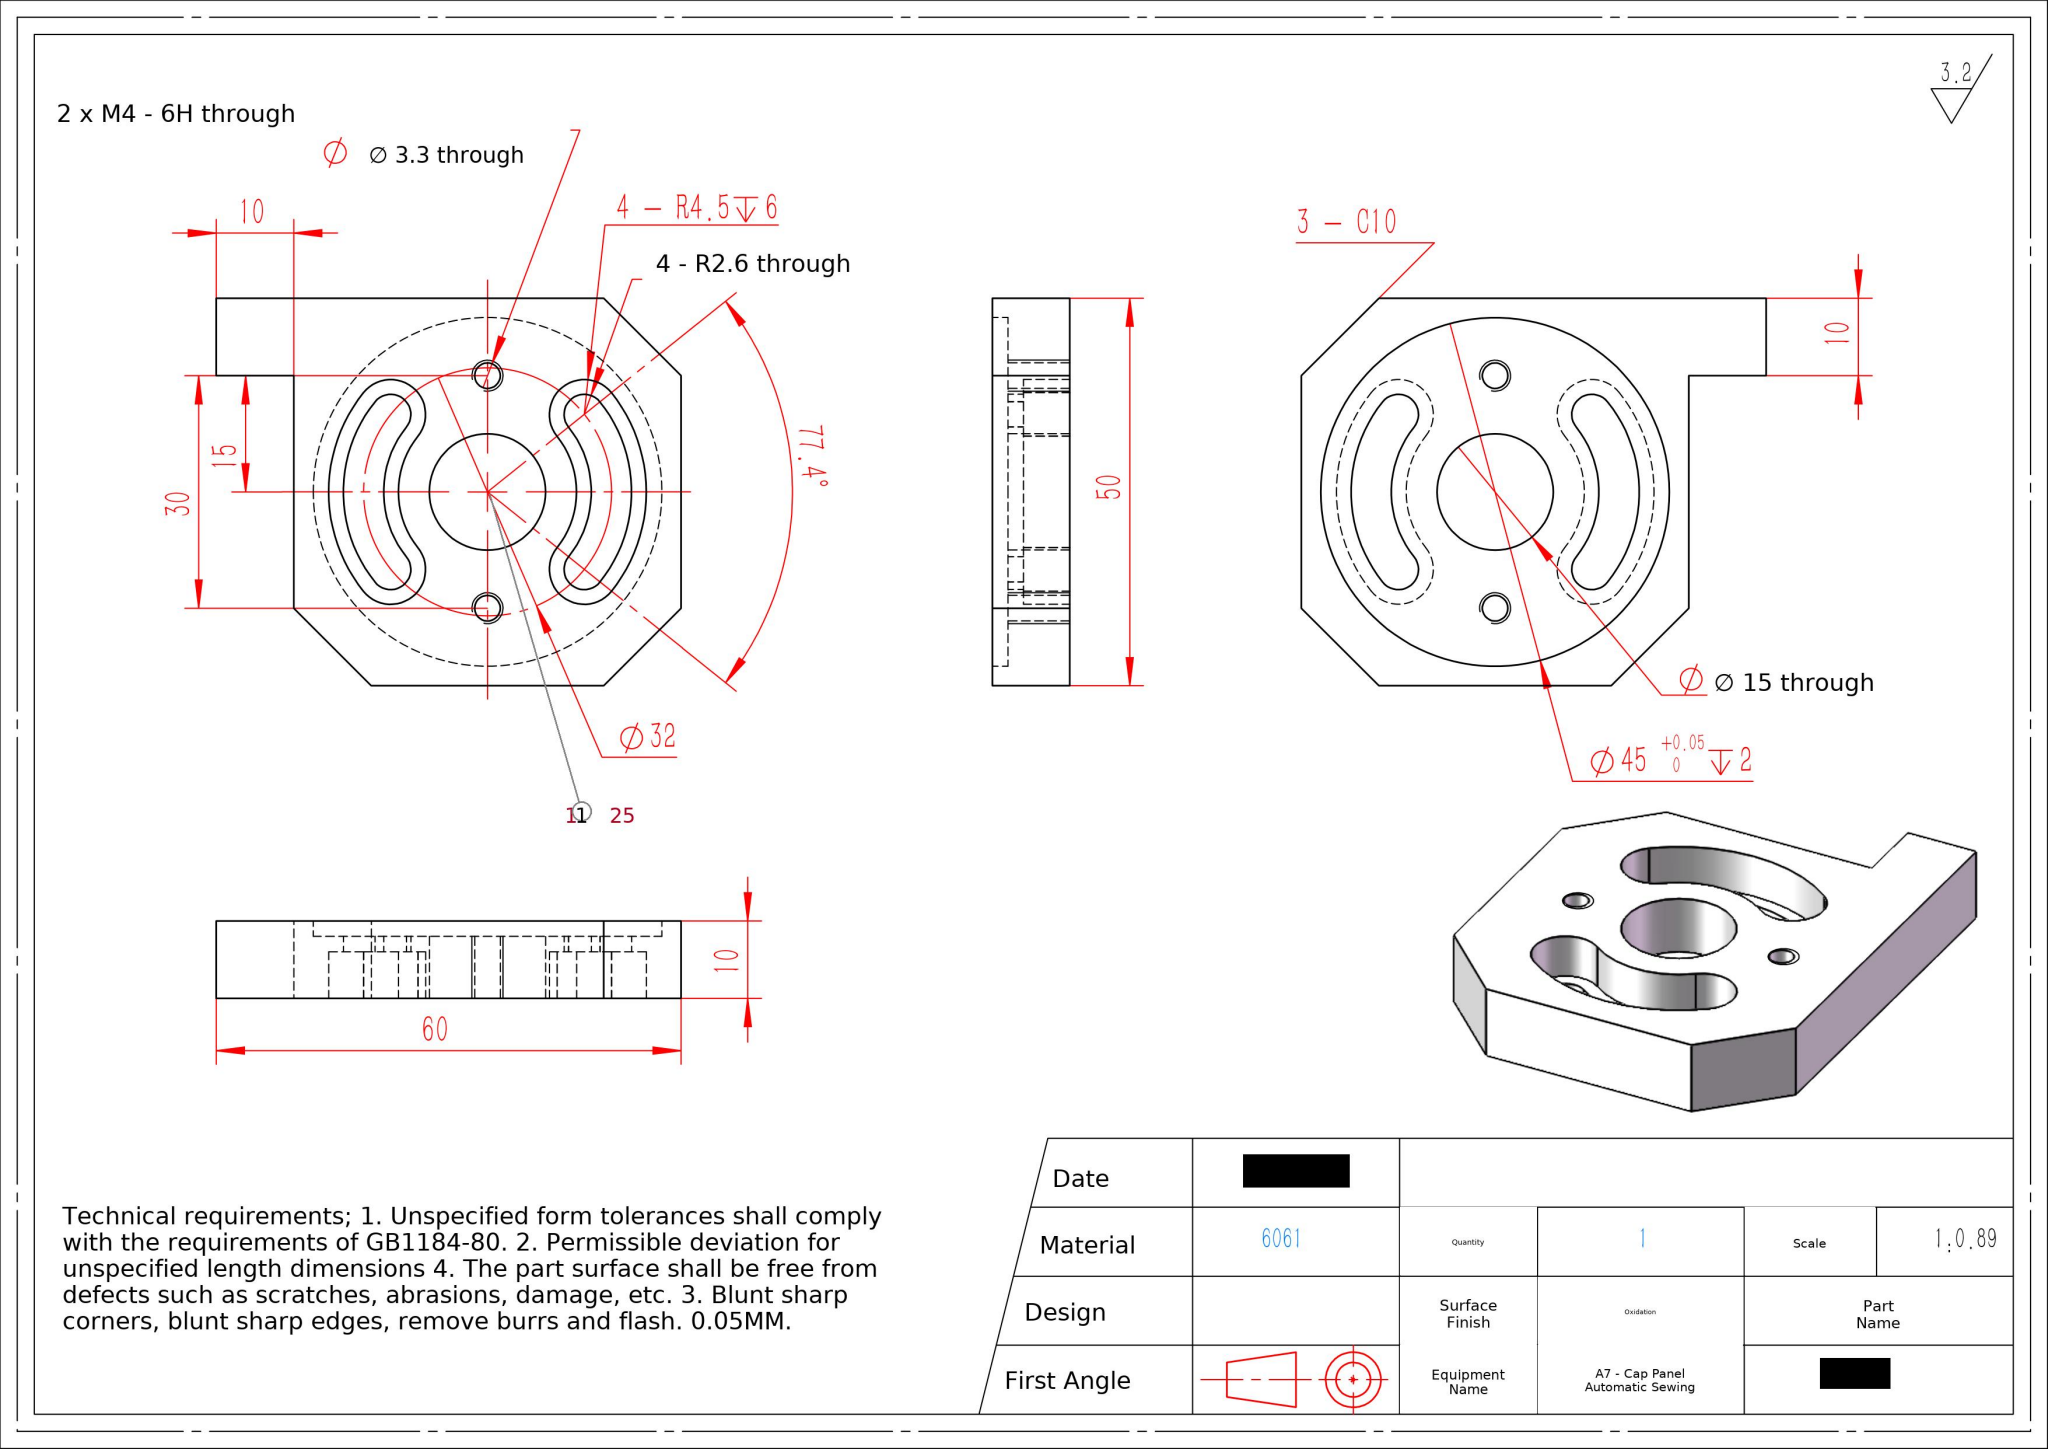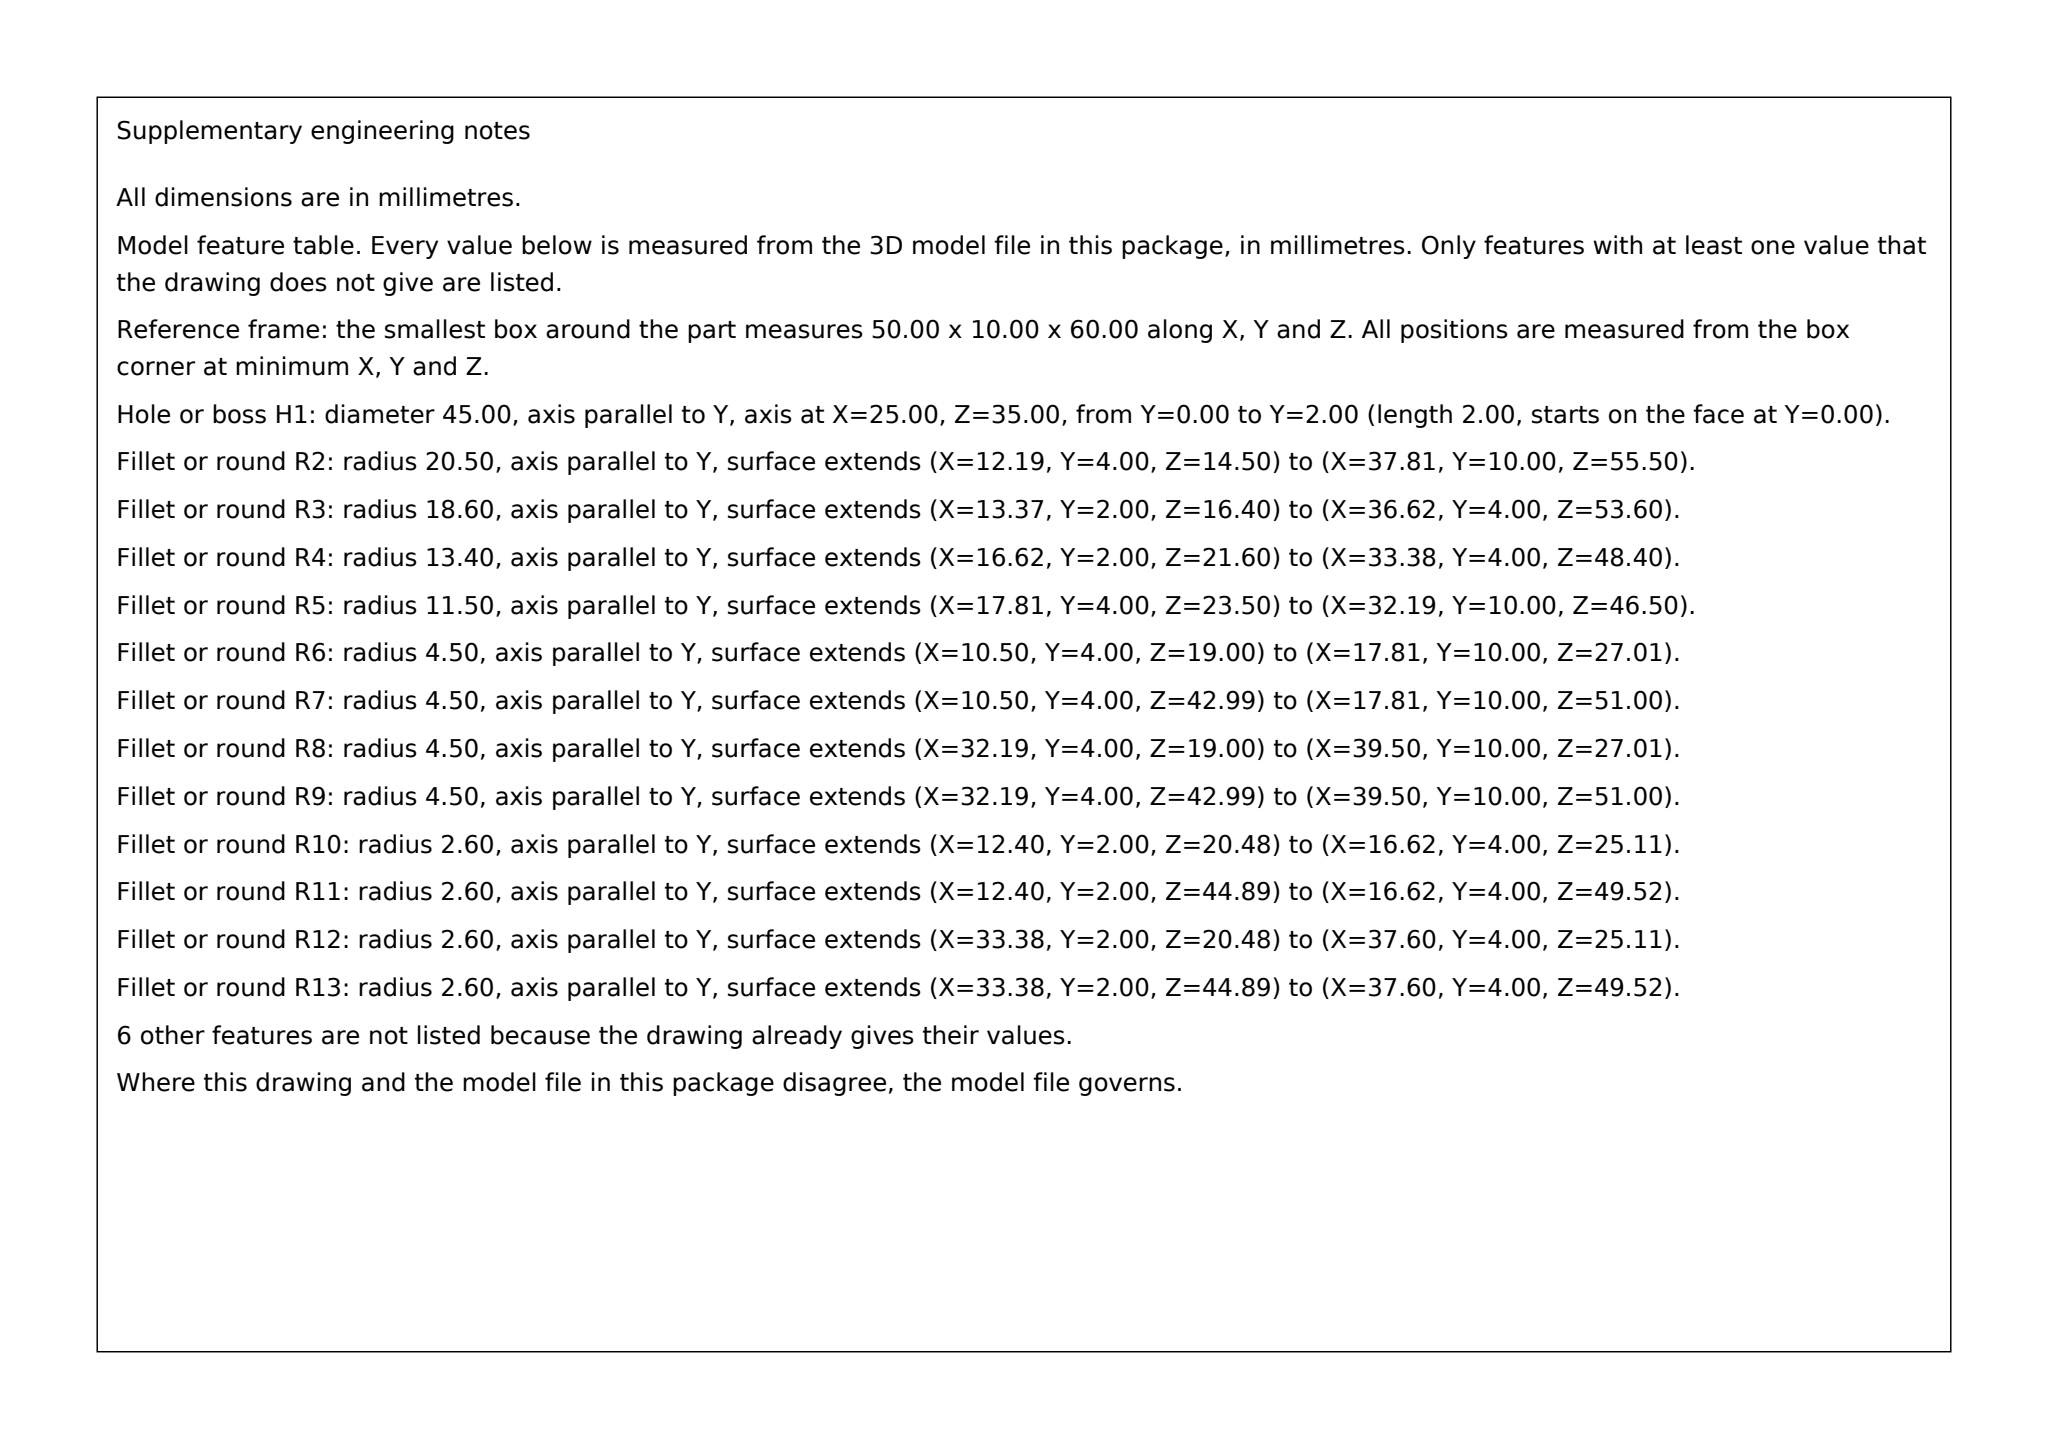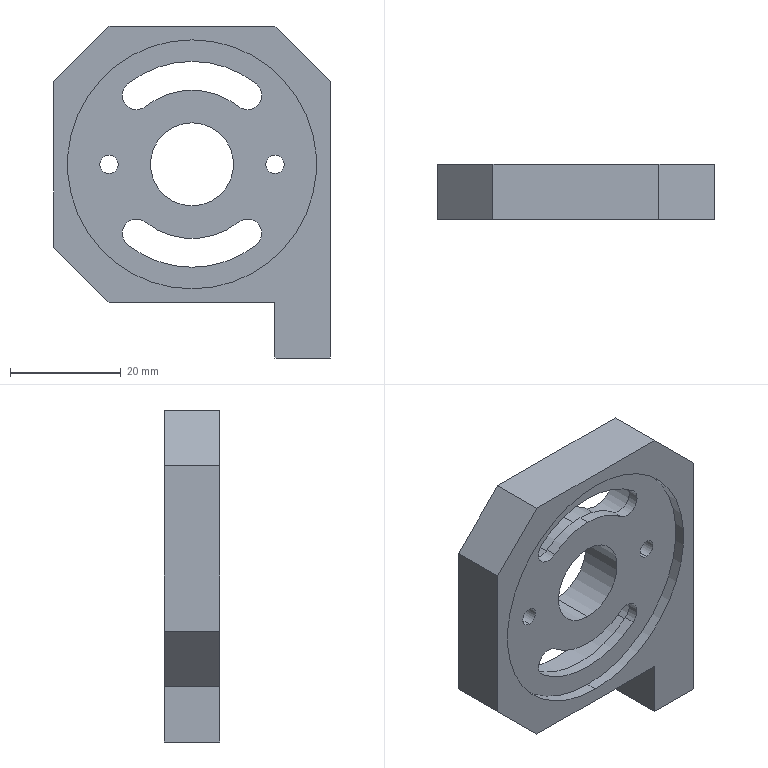Part | SolidWorks | mm | material 6061 | 1 solid | 46 faces | box 50 x 10 x 60 mm | volume 16138 mm3 | cylinder 32 | plane 14 | commonest cylinder face diameters 9 x6 5.2 x6 3.3 x4 41 x3 23 x3 37.2 x3 26.8 x3 45 x2
build123d program:
from build123d import *

# Parameters (mm, degrees)
SKETCH1_W           = 50
SKETCH1_H           = 50
BOSS_EXTRUDE1_DEPTH = 10
SKETCH2_R           = 7.5
CUT_EXTRUDE1_DEPTH  = 37.742
M4_TAPPED_HOLE1_D   = 3.3
SKETCH4_R           = 22.5
CUT_EXTRUDE2_DEPTH  = 2
CUT_EXTRUDE3_DEPTH  = 37.742
CUT_EXTRUDE4_DEPTH  = 6
SKETCH10_W          = 10
SKETCH10_H          = 10
BOSS_EXTRUDE2_DEPTH = 10
CHAMFER1_SIZE       = 10


with BuildPart() as part:
    # Sketch1 → Boss-Extrude1 (new body)
    with BuildSketch(Plane(origin=(0, 0, 0), x_dir=(1, 0, 0), z_dir=(0, 1, 0))):
        Rectangle(SKETCH1_W, SKETCH1_H)
    extrude(amount=BOSS_EXTRUDE1_DEPTH)

    # Sketch2 → Cut-Extrude1 (cut, through all)
    with BuildSketch(Plane(origin=(0, 10, 0), x_dir=(1, 0, 0), z_dir=(0, 1, 0))):
        with Locations(Location((0, 0, 0), (0, 0, 270))):
            Circle(SKETCH2_R)
    extrude(amount=-CUT_EXTRUDE1_DEPTH, mode=Mode.SUBTRACT)

    # M4 Tapped Hole1 (through all)
    with Locations(Plane(origin=(15, 10, 0), x_dir=(0, 0, 1), z_dir=(0, 1, 0))):
        with Locations((0, 0)):
            m4_tapped_hole1 = Hole(M4_TAPPED_HOLE1_D / 2)

    # Mirror1: M4 Tapped Hole1 across plane
    add(m4_tapped_hole1.mirror(Plane(origin=(0, 0, 0), x_dir=(0, 0, 1), z_dir=(1, 0, 0))), mode=Mode.SUBTRACT)

    # Sketch4 → Cut-Extrude2 (cut)
    with BuildSketch(Plane(origin=(0, 0, 0), x_dir=(-1, 0, 0), z_dir=(0, -1, 0))):
        with Locations(Location((0, 0, 0), (0, 0, 90))):
            Circle(SKETCH4_R)
    extrude(amount=-CUT_EXTRUDE2_DEPTH, mode=Mode.SUBTRACT)

    # Sketch5 → Cut-Extrude3 (cut, through all)
    with BuildSketch(Plane(origin=(0, 10, 0), x_dir=(1, 0, 0), z_dir=(0, 1, 0))):
        with BuildLine():
            ThreePointArc((-11.625, -14.52), (0, -18.6), (11.625, -14.52))
            ThreePointArc((11.625, -14.52), (12.03, -10.865), (8.375, -10.46))
            ThreePointArc((8.375, -10.46), (0, -13.4), (-8.375, -10.46))
            ThreePointArc((-8.375, -10.46), (-12.03, -10.865), (-11.625, -14.52))
        make_face()
    cut_extrude3 = extrude(amount=-CUT_EXTRUDE3_DEPTH, mode=Mode.SUBTRACT)

    # Sketch6 → Cut-Extrude4 (cut)
    with BuildSketch(Plane(origin=(0, 10, 0), x_dir=(1, 0, 0), z_dir=(0, 1, 0))):
        with BuildLine():
            ThreePointArc((-12.812, -16.003), (0, -20.5), (12.812, -16.003))
            ThreePointArc((12.812, -16.003), (13.513, -9.677), (7.188, -8.977))
            ThreePointArc((7.188, -8.977), (0, -11.5), (-7.188, -8.977))
            ThreePointArc((-7.188, -8.977), (-13.513, -9.677), (-12.812, -16.003))
        make_face()
    cut_extrude4 = extrude(amount=-CUT_EXTRUDE4_DEPTH, mode=Mode.SUBTRACT)

    # Mirror2: Cut-Extrude3, Cut-Extrude4 across plane
    add(cut_extrude3.mirror(Plane.XY), mode=Mode.SUBTRACT)
    add(cut_extrude4.mirror(Plane.XY), mode=Mode.SUBTRACT)

    # Sketch10 → Boss-Extrude2 (add)
    with BuildSketch(Plane(origin=(0, 0, -25), x_dir=(-1, 0, 0), z_dir=(0, 0, -1))):
        with Locations((-20, 5)):
            Rectangle(SKETCH10_W, SKETCH10_H)
    extrude(amount=BOSS_EXTRUDE2_DEPTH)

    # Chamfer1
    chamfer1_edges = [part.edges().sort_by_distance(p)[0] for p in [
        (25, 5, 25),
        (-25, 5, 25),
        (-25, 5, -25),
    ]]
    chamfer(chamfer1_edges, length=CHAMFER1_SIZE)


solid = part.part